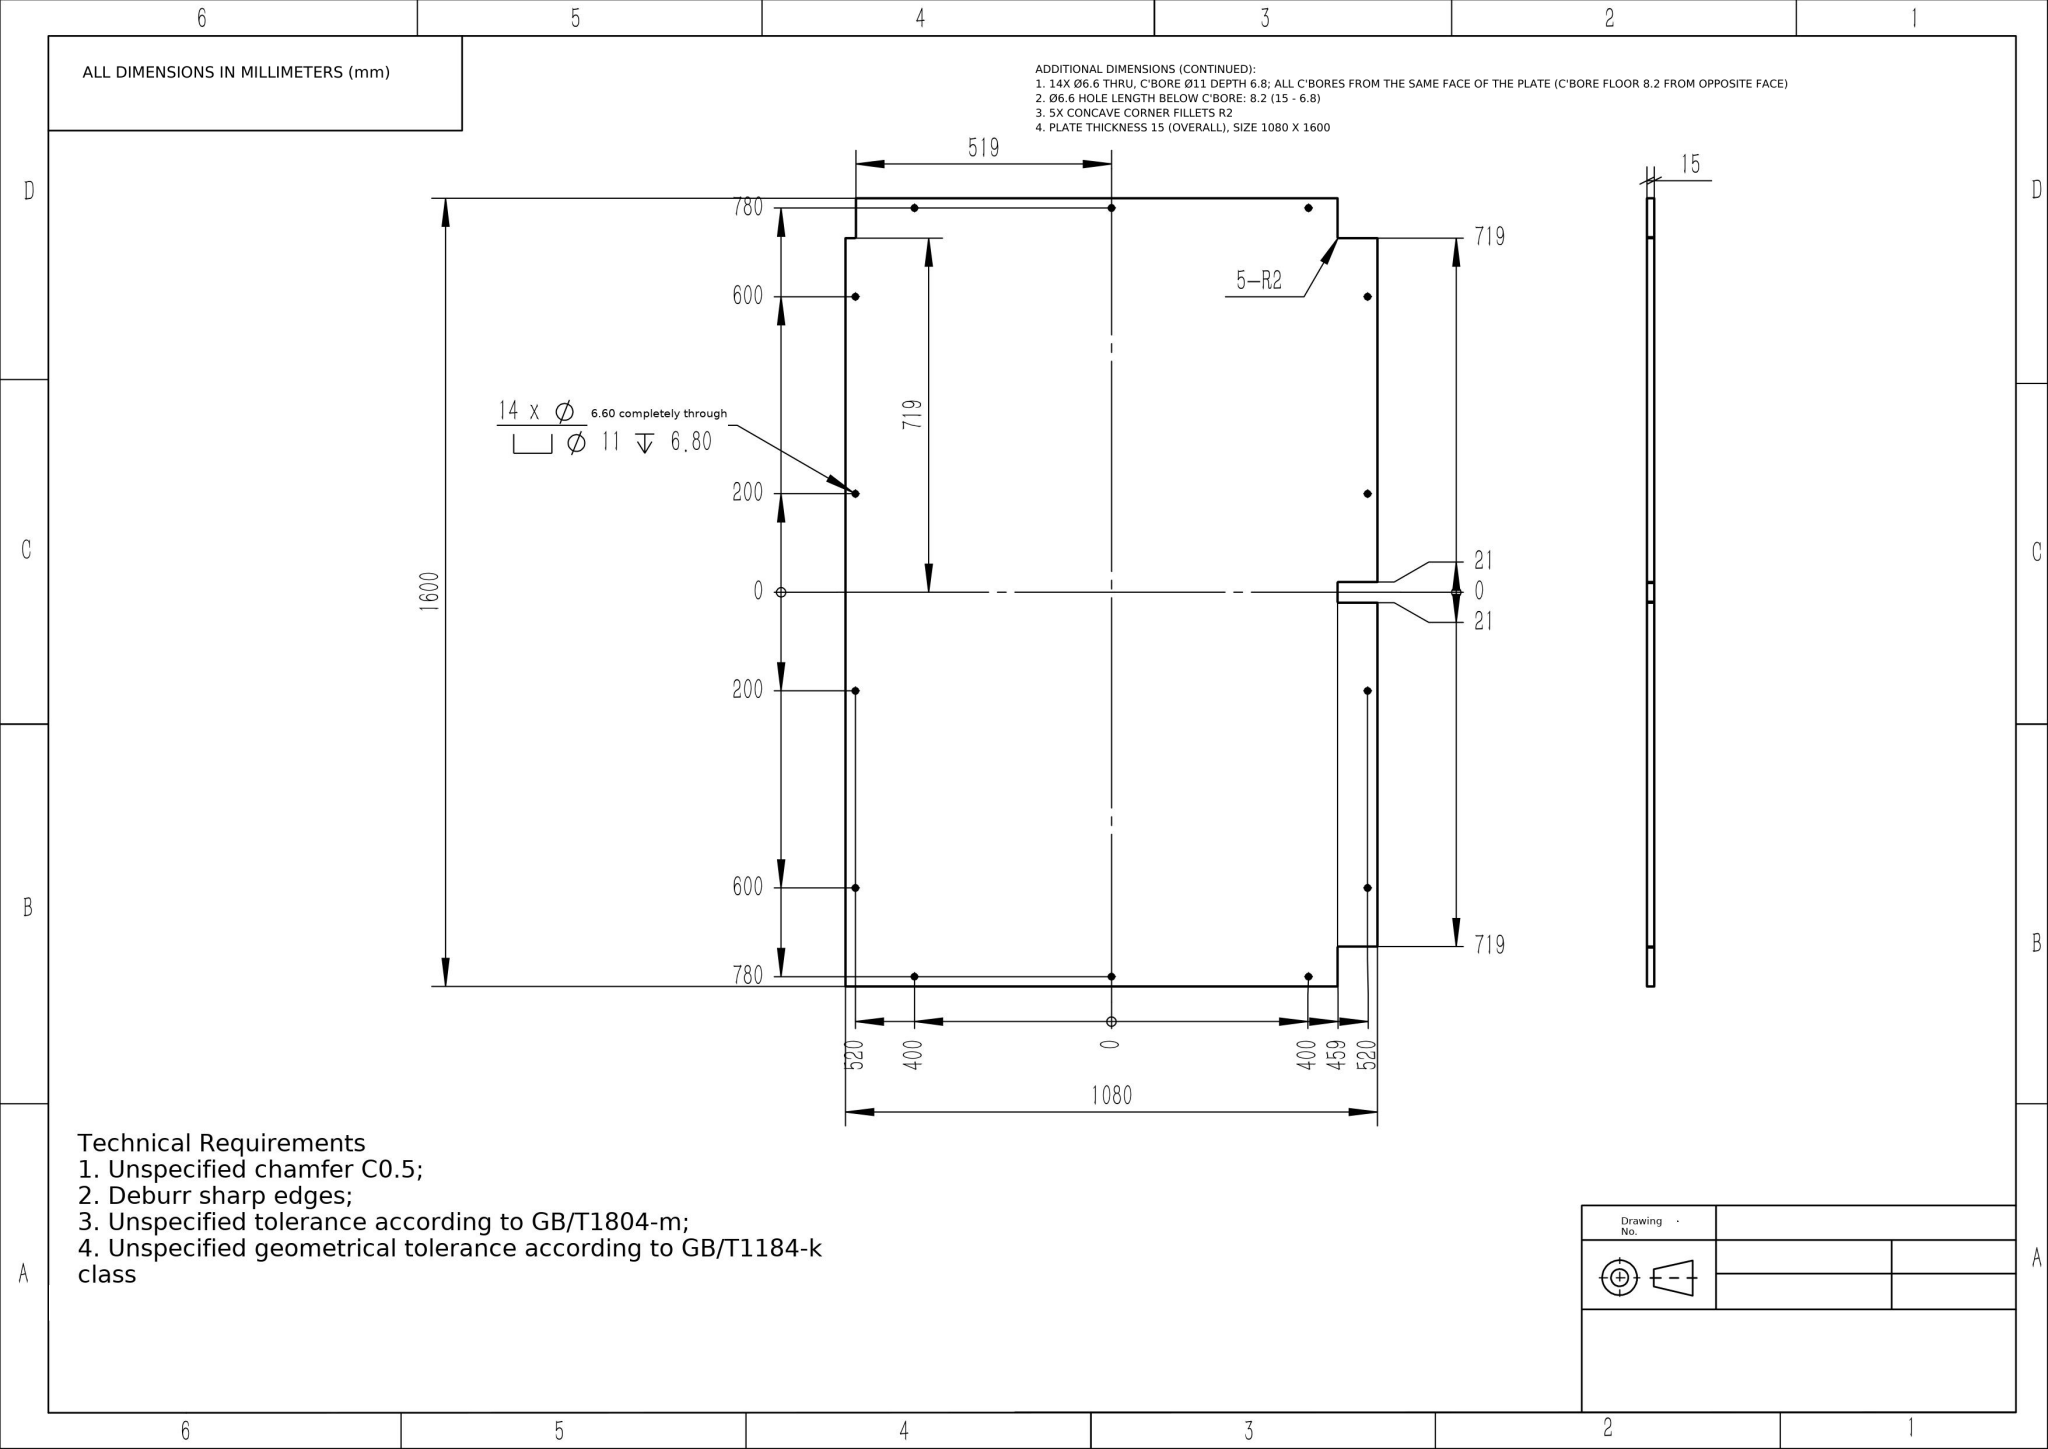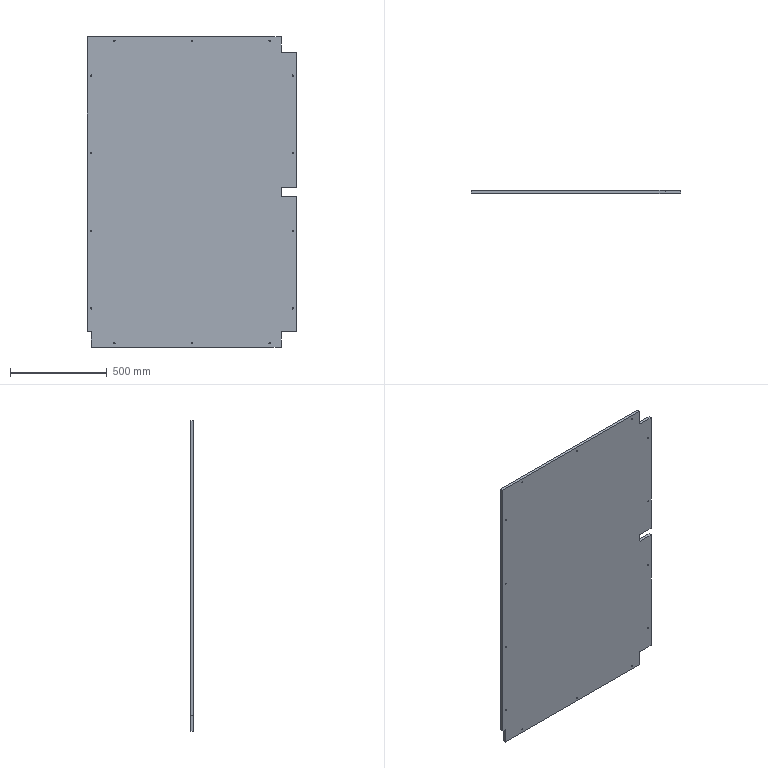Part | NX | mm | 1 solid | 91 faces | box 1080 x 15 x 1600 mm | volume 25633715 mm3 | cylinder 61 | plane 30 | commonest cylinder face diameters 11 x28 6.6 x28 4 x5